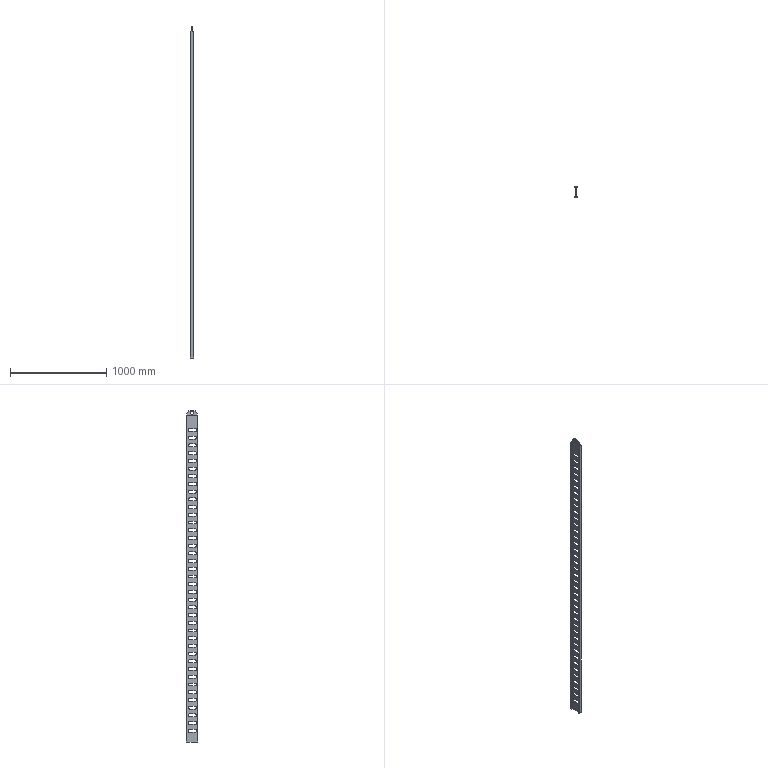Component | NX | REAR_BEAM | 1 solid | 181 faces | volume 1957422 mm3 | plane 99 | cylinder 82 | commonest cylinder face diameters 30 x81 110 x1